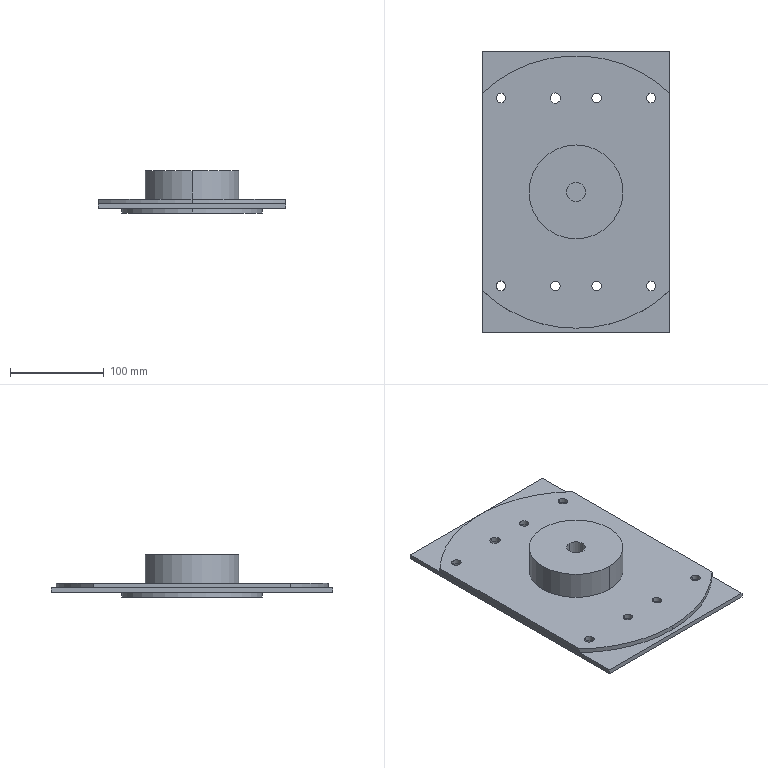Component | SolidWorks | FrontWheelAssembly-1_FrontWheelAccessory1-1 | 2 solids | 54 faces | box 200 x 300 x 45 mm | volume 872125 mm3 | cylinder 41 | plane 13 | commonest cylinder face diameters 10 x26 11.013 x4 290 x3 150 x2 20 x2 100 x2 10.462 x2
build123d program:
from build123d import *

# Parameters (mm, degrees)
SKETCH1_W           = 300
SKETCH1_H           = 200
BOSS_EXTRUDE1_DEPTH = 5
SKETCH2_R           = 75
BOSS_EXTRUDE2_DEPTH = 5
SKETCH6_R           = 5
CUT_EXTRUDE1_DEPTH  = 89
SKETCH7_R           = 5.231
SKETCH7_R_2         = 5
BOSS_EXTRUDE5_DEPTH = 5
SKETCH8_R           = 50
BOSS_EXTRUDE6_DEPTH = 30
SKETCH9_R           = 10
CUT_EXTRUDE2_DEPTH  = 33
SKETCH11_R          = 5
SKETCH11_R_2        = 5.507
CUT_EXTRUDE3_DEPTH  = 25
SKETCH12_R          = 5
CUT_EXTRUDE4_DEPTH  = 65


with BuildPart() as part:
    # Sketch1 → Boss-Extrude1 (new body)
    with BuildSketch(Plane.XY):
        Rectangle(SKETCH1_W, SKETCH1_H)
    extrude(amount=BOSS_EXTRUDE1_DEPTH)

    # Sketch2 → Boss-Extrude2 (add)
    with BuildSketch(Plane(origin=(0, 0, 0), x_dir=(-1, 0, 0), z_dir=(0, 0, -1))):
        Circle(SKETCH2_R)
    extrude(amount=BOSS_EXTRUDE2_DEPTH)

    # Sketch6 → Cut-Extrude1 (cut)
    with BuildSketch(Plane.XY.offset(5)):
        with Locations((-100, 80)):
            Circle(SKETCH6_R)
        with Locations((100, 80)):
            Circle(SKETCH6_R)
        with Locations((-100, -80)):
            Circle(SKETCH6_R)
        with Locations((100, -80)):
            Circle(SKETCH6_R)
    extrude(amount=-CUT_EXTRUDE1_DEPTH, mode=Mode.SUBTRACT)


with BuildPart() as body_2:
    # Sketch7 → Boss-Extrude5 (new body)
    with BuildSketch(Plane.XY.offset(5)):
        with BuildLine():
            Line((-105, 100), (105, 100))
            ThreePointArc((105, 100), (145, 0), (105, -100))
            Line((105, -100), (-105, -100))
            ThreePointArc((-105, -100), (-145, 0), (-105, 100))
        make_face()
        with Locations((-100, 80)):
            Circle(SKETCH7_R, mode=Mode.SUBTRACT)
        with Locations((100, 80)):
            Circle(SKETCH7_R_2, mode=Mode.SUBTRACT)
        with Locations((100, -80)):
            Circle(SKETCH7_R_2, mode=Mode.SUBTRACT)
        with Locations((-100, -80)):
            Circle(SKETCH7_R_2, mode=Mode.SUBTRACT)
    extrude(amount=BOSS_EXTRUDE5_DEPTH)

    # Sketch8 → Boss-Extrude6 (add)
    with BuildSketch(Plane.XY.offset(10)):
        Circle(SKETCH8_R)
    extrude(amount=BOSS_EXTRUDE6_DEPTH)

    # Sketch9 → Cut-Extrude2 (cut)
    with BuildSketch(Plane.XY.offset(40)):
        Circle(SKETCH9_R)
    extrude(amount=-CUT_EXTRUDE2_DEPTH, mode=Mode.SUBTRACT)


with BuildPart() as cut_extrude3_tool:
    # Sketch11 → Cut-Extrude3 (new body)
    with BuildSketch(Plane(origin=(0, 0, 0), x_dir=(-1, 0, 0), z_dir=(0, 0, -1))):
        with Locations(Location((-100, -22, 0), (0, 0, 180))):
            Circle(SKETCH11_R)
        with Locations(Location((-100, 22, 0), (0, 0, 180))):
            Circle(SKETCH11_R_2)
    extrude(amount=-CUT_EXTRUDE3_DEPTH)


with BuildPart() as part_1:
    add(part.part)

    # Cut-Extrude3: cut by cut_extrude3_tool
    add(cut_extrude3_tool.part, mode=Mode.SUBTRACT)


with BuildPart() as body_2_1:
    add(body_2.part)

    # Cut-Extrude3: cut by cut_extrude3_tool
    add(cut_extrude3_tool.part, mode=Mode.SUBTRACT)


with BuildPart() as cut_extrude4_tool:
    # Sketch12 → Cut-Extrude4 (new body)
    with BuildSketch(Plane(origin=(0, 0, 0), x_dir=(-1, 0, 0), z_dir=(0, 0, -1))):
        with Locations(Location((100, 22, 0), (0, 0, 180))):
            Circle(SKETCH12_R)
        with Locations(Location((100, -22, 0), (0, 0, 180))):
            Circle(SKETCH12_R)
    extrude(amount=-CUT_EXTRUDE4_DEPTH)


with BuildPart() as part_2:
    add(part_1.part)

    # Cut-Extrude4: cut by cut_extrude4_tool
    add(cut_extrude4_tool.part, mode=Mode.SUBTRACT)


with BuildPart() as body_2_2:
    add(body_2_1.part)

    # Cut-Extrude4: cut by cut_extrude4_tool
    add(cut_extrude4_tool.part, mode=Mode.SUBTRACT)


solid = Compound([part_2.part, body_2_2.part])

# Placed as in the assembly
solid = solid.moved(Location((25.629, -64.9, 228), (0, 0, 90)))